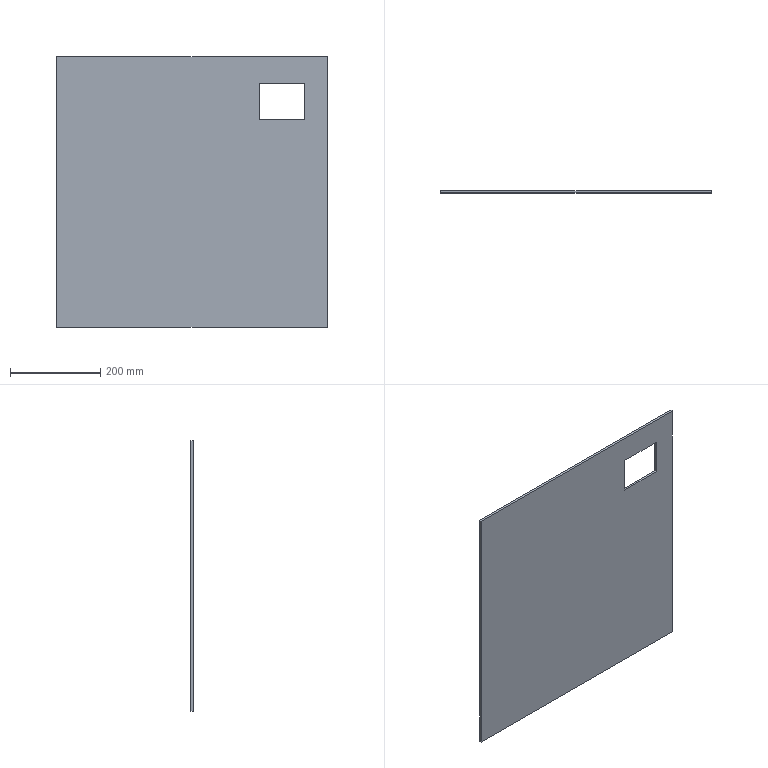Component | SolidWorks | CoverPlate3-1 | 1 solid | 10 faces | box 600 x 5 x 600 mm | volume 1760000 mm3 | plane 10
build123d program:
from build123d import *

# Parameters (mm, degrees)
SKETCH1_W      = 600
SKETCH1_H      = 600
EXTRUDE1_DEPTH = 5
SKETCH2_W      = 100
SKETCH2_H      = 80
EXTRUDE2_DEPTH = 5


with BuildPart() as part:
    # Sketch1 → Extrude1 (new body)
    with BuildSketch(Plane.XY):
        Rectangle(SKETCH1_W, SKETCH1_H)
    extrude(amount=EXTRUDE1_DEPTH)

    # Sketch2 → Extrude2 (cut)
    with BuildSketch(Plane.XY.offset(5)):
        with Locations((200, -200)):
            Rectangle(SKETCH2_W, SKETCH2_H)
    extrude(amount=-EXTRUDE2_DEPTH, mode=Mode.SUBTRACT)


solid = part.part

# Placed as in the assembly
solid = solid.moved(Location((0, -165, 280), (-90, 0, 0)))
STEP:
#1=COLOUR_RGB('',0.7922,0.8196,0.9333);
#2=FILL_AREA_STYLE_COLOUR('',#1);
#3=FILL_AREA_STYLE('',(#2));
#4=SURFACE_STYLE_FILL_AREA(#3);
#5=SURFACE_SIDE_STYLE('',(#4));
#6=SURFACE_STYLE_USAGE(.BOTH.,#5);
#7=PRESENTATION_STYLE_ASSIGNMENT((#6));
#8=CARTESIAN_POINT('',(11.811,-6.496,22.835));
#9=VERTEX_POINT('',#8);
#10=CARTESIAN_POINT('',(11.811,-6.496,-0.7874));
#11=VERTEX_POINT('',#10);
#12=CARTESIAN_POINT('',(11.811,-6.496,-0.7874));
#13=DIRECTION('',(-0.,0.,-1.));
#14=VECTOR('',#13,39.37);
#15=LINE('',#12,#14);
#16=EDGE_CURVE('',#9,#11,#15,.T.);
#17=ORIENTED_EDGE('',*,*,#16,.T.);
#18=CARTESIAN_POINT('',(11.811,-6.299,-0.7874));
#19=VERTEX_POINT('',#18);
#20=CARTESIAN_POINT('',(11.811,-6.299,-0.7874));
#21=DIRECTION('',(0.,-1.,0.));
#22=VECTOR('',#21,39.37);
#23=LINE('',#20,#22);
#24=EDGE_CURVE('',#19,#11,#23,.T.);
#25=ORIENTED_EDGE('',*,*,#24,.F.);
#26=CARTESIAN_POINT('',(11.811,-6.299,22.835));
#27=VERTEX_POINT('',#26);
#28=CARTESIAN_POINT('',(11.811,-6.299,-0.7874));
#29=DIRECTION('',(-0.,0.,-1.));
#30=VECTOR('',#29,39.37);
#31=LINE('',#28,#30);
#32=EDGE_CURVE('',#27,#19,#31,.T.);
#33=ORIENTED_EDGE('',*,*,#32,.F.);
#34=CARTESIAN_POINT('',(11.811,-6.299,22.835));
#35=DIRECTION('',(0.,-1.,0.));
#36=VECTOR('',#35,39.37);
#37=LINE('',#34,#36);
#38=EDGE_CURVE('',#27,#9,#37,.T.);
#39=ORIENTED_EDGE('',*,*,#38,.T.);
#40=EDGE_LOOP('',(#17,#25,#33,#39));
#41=FACE_OUTER_BOUND('',#40,.T.);
#42=CARTESIAN_POINT('',(11.811,-6.299,-0.7874));
#43=DIRECTION('',(-1.,0.,0.));
#44=DIRECTION('',(0.,0.,1.));
#45=AXIS2_PLACEMENT_3D('',#42,#43,#44);
#46=PLANE('',#45);
#47=ADVANCED_FACE('',(#41),#46,.F.);
#48=CARTESIAN_POINT('',(-11.811,-6.496,-0.7874));
#49=VERTEX_POINT('',#48);
#50=CARTESIAN_POINT('',(-11.811,-6.496,-0.7874));
#51=DIRECTION('',(-1.,0.,0.));
#52=VECTOR('',#51,39.37);
#53=LINE('',#50,#52);
#54=EDGE_CURVE('',#11,#49,#53,.T.);
#55=ORIENTED_EDGE('',*,*,#54,.T.);
#56=CARTESIAN_POINT('',(-11.811,-6.299,-0.7874));
#57=VERTEX_POINT('',#56);
#58=CARTESIAN_POINT('',(-11.811,-6.299,-0.7874));
#59=DIRECTION('',(0.,-1.,0.));
#60=VECTOR('',#59,39.37);
#61=LINE('',#58,#60);
#62=EDGE_CURVE('',#57,#49,#61,.T.);
#63=ORIENTED_EDGE('',*,*,#62,.F.);
#64=CARTESIAN_POINT('',(-11.811,-6.299,-0.7874));
#65=DIRECTION('',(-1.,0.,0.));
#66=VECTOR('',#65,39.37);
#67=LINE('',#64,#66);
#68=EDGE_CURVE('',#19,#57,#67,.T.);
#69=ORIENTED_EDGE('',*,*,#68,.F.);
#70=ORIENTED_EDGE('',*,*,#24,.T.);
#71=EDGE_LOOP('',(#55,#63,#69,#70));
#72=FACE_OUTER_BOUND('',#71,.T.);
#73=CARTESIAN_POINT('',(-11.811,-6.299,-0.7874));
#74=DIRECTION('',(0.,0.,1.));
#75=DIRECTION('',(0.,-1.,0.));
#76=AXIS2_PLACEMENT_3D('',#73,#74,#75);
#77=PLANE('',#76);
#78=ADVANCED_FACE('',(#72),#77,.F.);
#79=CARTESIAN_POINT('',(-11.811,-6.496,22.835));
#80=VERTEX_POINT('',#79);
#81=CARTESIAN_POINT('',(-11.811,-6.496,-0.7874));
#82=DIRECTION('',(0.,0.,1.));
#83=VECTOR('',#82,39.37);
#84=LINE('',#81,#83);
#85=EDGE_CURVE('',#49,#80,#84,.T.);
#86=ORIENTED_EDGE('',*,*,#85,.T.);
#87=CARTESIAN_POINT('',(-11.811,-6.299,22.835));
#88=VERTEX_POINT('',#87);
#89=CARTESIAN_POINT('',(-11.811,-6.299,22.835));
#90=DIRECTION('',(0.,-1.,0.));
#91=VECTOR('',#90,39.37);
#92=LINE('',#89,#91);
#93=EDGE_CURVE('',#88,#80,#92,.T.);
#94=ORIENTED_EDGE('',*,*,#93,.F.);
#95=CARTESIAN_POINT('',(-11.811,-6.299,-0.7874));
#96=DIRECTION('',(0.,0.,1.));
#97=VECTOR('',#96,39.37);
#98=LINE('',#95,#97);
#99=EDGE_CURVE('',#57,#88,#98,.T.);
#100=ORIENTED_EDGE('',*,*,#99,.F.);
#101=ORIENTED_EDGE('',*,*,#62,.T.);
#102=EDGE_LOOP('',(#86,#94,#100,#101));
#103=FACE_OUTER_BOUND('',#102,.T.);
#104=CARTESIAN_POINT('',(-11.811,-6.299,-0.7874));
#105=DIRECTION('',(1.,0.,-0.));
#106=DIRECTION('',(-0.,0.,-1.));
#107=AXIS2_PLACEMENT_3D('',#104,#105,#106);
#108=PLANE('',#107);
#109=ADVANCED_FACE('',(#103),#108,.F.);
#110=CARTESIAN_POINT('',(-11.811,-6.496,22.835));
#111=DIRECTION('',(1.,0.,0.));
#112=VECTOR('',#111,39.37);
#113=LINE('',#110,#112);
#114=EDGE_CURVE('',#80,#9,#113,.T.);
#115=ORIENTED_EDGE('',*,*,#114,.T.);
#116=ORIENTED_EDGE('',*,*,#38,.F.);
#117=CARTESIAN_POINT('',(-11.811,-6.299,22.835));
#118=DIRECTION('',(1.,0.,0.));
#119=VECTOR('',#118,39.37);
#120=LINE('',#117,#119);
#121=EDGE_CURVE('',#88,#27,#120,.T.);
#122=ORIENTED_EDGE('',*,*,#121,.F.);
#123=ORIENTED_EDGE('',*,*,#93,.T.);
#124=EDGE_LOOP('',(#115,#116,#122,#123));
#125=FACE_OUTER_BOUND('',#124,.T.);
#126=CARTESIAN_POINT('',(-11.811,-6.299,22.835));
#127=DIRECTION('',(0.,0.,-1.));
#128=DIRECTION('',(0.,1.,0.));
#129=AXIS2_PLACEMENT_3D('',#126,#127,#128);
#130=PLANE('',#129);
#131=ADVANCED_FACE('',(#125),#130,.F.);
#132=CARTESIAN_POINT('',(9.843,-6.299,20.472));
#133=VERTEX_POINT('',#132);
#134=CARTESIAN_POINT('',(9.843,-6.299,17.323));
#135=VERTEX_POINT('',#134);
#136=CARTESIAN_POINT('',(9.843,-6.299,17.323));
#137=DIRECTION('',(-0.,0.,-1.));
#138=VECTOR('',#137,39.37);
#139=LINE('',#136,#138);
#140=EDGE_CURVE('',#133,#135,#139,.T.);
#141=ORIENTED_EDGE('',*,*,#140,.F.);
#142=CARTESIAN_POINT('',(5.906,-6.299,20.472));
#143=VERTEX_POINT('',#142);
#144=CARTESIAN_POINT('',(5.906,-6.299,20.472));
#145=DIRECTION('',(1.,0.,0.));
#146=VECTOR('',#145,39.37);
#147=LINE('',#144,#146);
#148=EDGE_CURVE('',#143,#133,#147,.T.);
#149=ORIENTED_EDGE('',*,*,#148,.F.);
#150=CARTESIAN_POINT('',(5.906,-6.299,17.323));
#151=VERTEX_POINT('',#150);
#152=CARTESIAN_POINT('',(5.906,-6.299,17.323));
#153=DIRECTION('',(0.,0.,1.));
#154=VECTOR('',#153,39.37);
#155=LINE('',#152,#154);
#156=EDGE_CURVE('',#151,#143,#155,.T.);
#157=ORIENTED_EDGE('',*,*,#156,.F.);
#158=CARTESIAN_POINT('',(5.906,-6.299,17.323));
#159=DIRECTION('',(-1.,0.,0.));
#160=VECTOR('',#159,39.37);
#161=LINE('',#158,#160);
#162=EDGE_CURVE('',#135,#151,#161,.T.);
#163=ORIENTED_EDGE('',*,*,#162,.F.);
#164=EDGE_LOOP('',(#141,#149,#157,#163));
#165=FACE_BOUND('',#164,.T.);
#166=ORIENTED_EDGE('',*,*,#32,.T.);
#167=ORIENTED_EDGE('',*,*,#68,.T.);
#168=ORIENTED_EDGE('',*,*,#99,.T.);
#169=ORIENTED_EDGE('',*,*,#121,.T.);
#170=EDGE_LOOP('',(#166,#167,#168,#169));
#171=FACE_OUTER_BOUND('',#170,.T.);
#172=CARTESIAN_POINT('',(0.,-6.299,11.024));
#173=DIRECTION('',(0.,1.,0.));
#174=DIRECTION('',(1.,0.,0.));
#175=AXIS2_PLACEMENT_3D('',#172,#173,#174);
#176=PLANE('',#175);
#177=ADVANCED_FACE('',(#165,#171),#176,.T.);
#178=CARTESIAN_POINT('',(5.906,-6.496,20.472));
#179=VERTEX_POINT('',#178);
#180=CARTESIAN_POINT('',(9.843,-6.496,20.472));
#181=VERTEX_POINT('',#180);
#182=CARTESIAN_POINT('',(5.906,-6.496,20.472));
#183=DIRECTION('',(1.,0.,0.));
#184=VECTOR('',#183,39.37);
#185=LINE('',#182,#184);
#186=EDGE_CURVE('',#179,#181,#185,.T.);
#187=ORIENTED_EDGE('',*,*,#186,.T.);
#188=CARTESIAN_POINT('',(9.843,-6.496,17.323));
#189=VERTEX_POINT('',#188);
#190=CARTESIAN_POINT('',(9.843,-6.496,17.323));
#191=DIRECTION('',(-0.,0.,-1.));
#192=VECTOR('',#191,39.37);
#193=LINE('',#190,#192);
#194=EDGE_CURVE('',#181,#189,#193,.T.);
#195=ORIENTED_EDGE('',*,*,#194,.T.);
#196=CARTESIAN_POINT('',(5.906,-6.496,17.323));
#197=VERTEX_POINT('',#196);
#198=CARTESIAN_POINT('',(5.906,-6.496,17.323));
#199=DIRECTION('',(-1.,0.,0.));
#200=VECTOR('',#199,39.37);
#201=LINE('',#198,#200);
#202=EDGE_CURVE('',#189,#197,#201,.T.);
#203=ORIENTED_EDGE('',*,*,#202,.T.);
#204=CARTESIAN_POINT('',(5.906,-6.496,17.323));
#205=DIRECTION('',(0.,0.,1.));
#206=VECTOR('',#205,39.37);
#207=LINE('',#204,#206);
#208=EDGE_CURVE('',#197,#179,#207,.T.);
#209=ORIENTED_EDGE('',*,*,#208,.T.);
#210=EDGE_LOOP('',(#187,#195,#203,#209));
#211=FACE_BOUND('',#210,.T.);
#212=ORIENTED_EDGE('',*,*,#16,.F.);
#213=ORIENTED_EDGE('',*,*,#114,.F.);
#214=ORIENTED_EDGE('',*,*,#85,.F.);
#215=ORIENTED_EDGE('',*,*,#54,.F.);
#216=EDGE_LOOP('',(#212,#213,#214,#215));
#217=FACE_OUTER_BOUND('',#216,.T.);
#218=CARTESIAN_POINT('',(0.,-6.496,11.024));
#219=DIRECTION('',(0.,1.,0.));
#220=DIRECTION('',(1.,0.,0.));
#221=AXIS2_PLACEMENT_3D('',#218,#219,#220);
#222=PLANE('',#221);
#223=ADVANCED_FACE('',(#211,#217),#222,.F.);
#224=ORIENTED_EDGE('',*,*,#140,.T.);
#225=CARTESIAN_POINT('',(9.843,-6.496,17.323));
#226=DIRECTION('',(0.,1.,0.));
#227=VECTOR('',#226,39.37);
#228=LINE('',#225,#227);
#229=EDGE_CURVE('',#189,#135,#228,.T.);
#230=ORIENTED_EDGE('',*,*,#229,.F.);
#231=ORIENTED_EDGE('',*,*,#194,.F.);
#232=CARTESIAN_POINT('',(9.843,-6.496,20.472));
#233=DIRECTION('',(0.,1.,0.));
#234=VECTOR('',#233,39.37);
#235=LINE('',#232,#234);
#236=EDGE_CURVE('',#181,#133,#235,.T.);
#237=ORIENTED_EDGE('',*,*,#236,.T.);
#238=EDGE_LOOP('',(#224,#230,#231,#237));
#239=FACE_OUTER_BOUND('',#238,.T.);
#240=CARTESIAN_POINT('',(9.843,-6.496,17.323));
#241=DIRECTION('',(1.,0.,-0.));
#242=DIRECTION('',(-0.,0.,-1.));
#243=AXIS2_PLACEMENT_3D('',#240,#241,#242);
#244=PLANE('',#243);
#245=ADVANCED_FACE('',(#239),#244,.F.);
#246=ORIENTED_EDGE('',*,*,#148,.T.);
#247=ORIENTED_EDGE('',*,*,#236,.F.);
#248=ORIENTED_EDGE('',*,*,#186,.F.);
#249=CARTESIAN_POINT('',(5.906,-6.496,20.472));
#250=DIRECTION('',(0.,1.,0.));
#251=VECTOR('',#250,39.37);
#252=LINE('',#249,#251);
#253=EDGE_CURVE('',#179,#143,#252,.T.);
#254=ORIENTED_EDGE('',*,*,#253,.T.);
#255=EDGE_LOOP('',(#246,#247,#248,#254));
#256=FACE_OUTER_BOUND('',#255,.T.);
#257=CARTESIAN_POINT('',(5.906,-6.496,20.472));
#258=DIRECTION('',(0.,0.,1.));
#259=DIRECTION('',(0.,-1.,0.));
#260=AXIS2_PLACEMENT_3D('',#257,#258,#259);
#261=PLANE('',#260);
#262=ADVANCED_FACE('',(#256),#261,.F.);
#263=ORIENTED_EDGE('',*,*,#156,.T.);
#264=ORIENTED_EDGE('',*,*,#253,.F.);
#265=ORIENTED_EDGE('',*,*,#208,.F.);
#266=CARTESIAN_POINT('',(5.906,-6.496,17.323));
#267=DIRECTION('',(0.,1.,0.));
#268=VECTOR('',#267,39.37);
#269=LINE('',#266,#268);
#270=EDGE_CURVE('',#197,#151,#269,.T.);
#271=ORIENTED_EDGE('',*,*,#270,.T.);
#272=EDGE_LOOP('',(#263,#264,#265,#271));
#273=FACE_OUTER_BOUND('',#272,.T.);
#274=CARTESIAN_POINT('',(5.906,-6.496,17.323));
#275=DIRECTION('',(-1.,0.,0.));
#276=DIRECTION('',(0.,1.,0.));
#277=AXIS2_PLACEMENT_3D('',#274,#275,#276);
#278=PLANE('',#277);
#279=ADVANCED_FACE('',(#273),#278,.F.);
#280=ORIENTED_EDGE('',*,*,#162,.T.);
#281=ORIENTED_EDGE('',*,*,#270,.F.);
#282=ORIENTED_EDGE('',*,*,#202,.F.);
#283=ORIENTED_EDGE('',*,*,#229,.T.);
#284=EDGE_LOOP('',(#280,#281,#282,#283));
#285=FACE_OUTER_BOUND('',#284,.T.);
#286=CARTESIAN_POINT('',(5.906,-6.496,17.323));
#287=DIRECTION('',(0.,0.,-1.));
#288=DIRECTION('',(0.,1.,0.));
#289=AXIS2_PLACEMENT_3D('',#286,#287,#288);
#290=PLANE('',#289);
#291=ADVANCED_FACE('',(#285),#290,.F.);
#292=CLOSED_SHELL('',(#47,#78,#109,#131,#177,#223,#245,#262,#279,#291));
#293=MANIFOLD_SOLID_BREP('',#292);
#294=STYLED_ITEM('',(#7),#293);
#295=PRESENTATION_LAYER_ASSIGNMENT('','',(#294));
#296=CARTESIAN_POINT('',(0.,0.,0.));
#297=DIRECTION('',(0.,0.,1.));
#298=DIRECTION('',(1.,0.,0.));
#299=AXIS2_PLACEMENT_3D('',#296,#297,#298);
#300=(LENGTH_UNIT()NAMED_UNIT(*)SI_UNIT($,.METRE.));
#301=LENGTH_MEASURE_WITH_UNIT(LENGTH_MEASURE(0.0254),#300);
#302=DIMENSIONAL_EXPONENTS(1.,0.,0.,0.,0.,0.,0.);
#303=(CONVERSION_BASED_UNIT('',#301)LENGTH_UNIT()NAMED_UNIT(#302));
#304=UNCERTAINTY_MEASURE_WITH_UNIT(LENGTH_MEASURE(0.00001),#303,'','');
#305=(NAMED_UNIT(*)PLANE_ANGLE_UNIT()SI_UNIT($,.RADIAN.));
#306=(NAMED_UNIT(*)SI_UNIT($,.STERADIAN.)SOLID_ANGLE_UNIT());
#307=(GEOMETRIC_REPRESENTATION_CONTEXT(3)GLOBAL_UNCERTAINTY_ASSIGNED_CONTEXT((#304))GLOBAL_UNIT_ASSIGNED_CONTEXT((#303,#305,#306))REPRESENTATION_CONTEXT('',''));
#308=ADVANCED_BREP_SHAPE_REPRESENTATION('',(#293,#299),#307);
#309=(LENGTH_UNIT()NAMED_UNIT(*)SI_UNIT($,.METRE.));
#310=LENGTH_MEASURE_WITH_UNIT(LENGTH_MEASURE(0.0254),#309);
#311=DIMENSIONAL_EXPONENTS(1.,0.,0.,0.,0.,0.,0.);
#312=(CONVERSION_BASED_UNIT('',#310)LENGTH_UNIT()NAMED_UNIT(#311));
#313=UNCERTAINTY_MEASURE_WITH_UNIT(LENGTH_MEASURE(0.00001),#312,'','');
#314=(NAMED_UNIT(*)PLANE_ANGLE_UNIT()SI_UNIT($,.RADIAN.));
#315=(NAMED_UNIT(*)SI_UNIT($,.STERADIAN.)SOLID_ANGLE_UNIT());
#316=(GEOMETRIC_REPRESENTATION_CONTEXT(3)GLOBAL_UNCERTAINTY_ASSIGNED_CONTEXT((#313))GLOBAL_UNIT_ASSIGNED_CONTEXT((#312,#314,#315))REPRESENTATION_CONTEXT('',''));
#317=MECHANICAL_DESIGN_GEOMETRIC_PRESENTATION_REPRESENTATION('',(#294),#316);